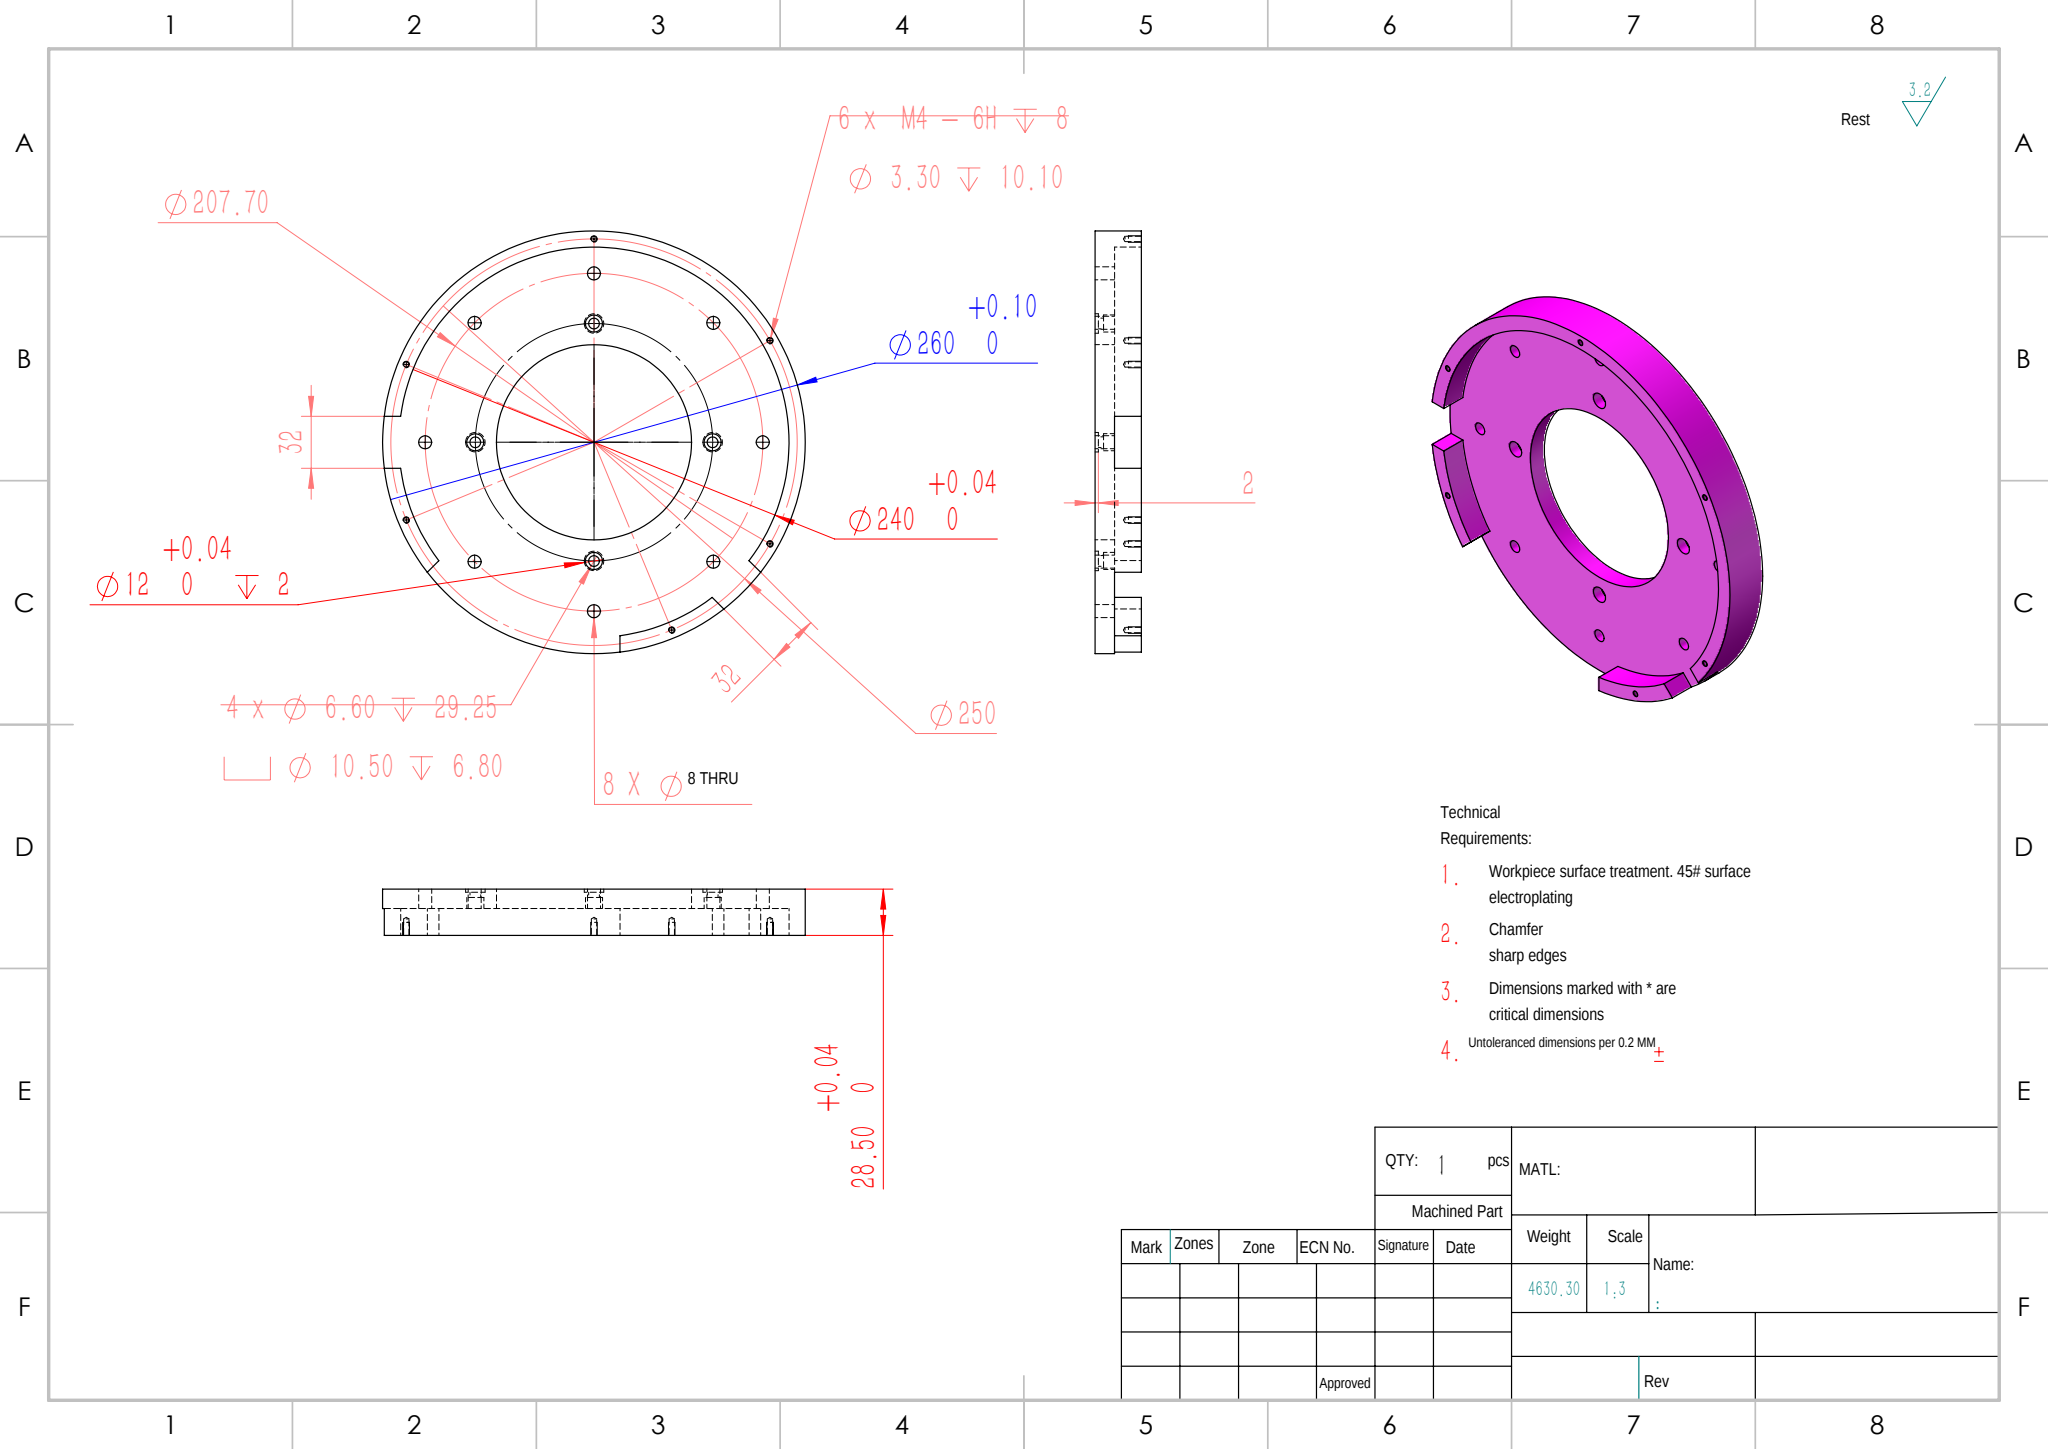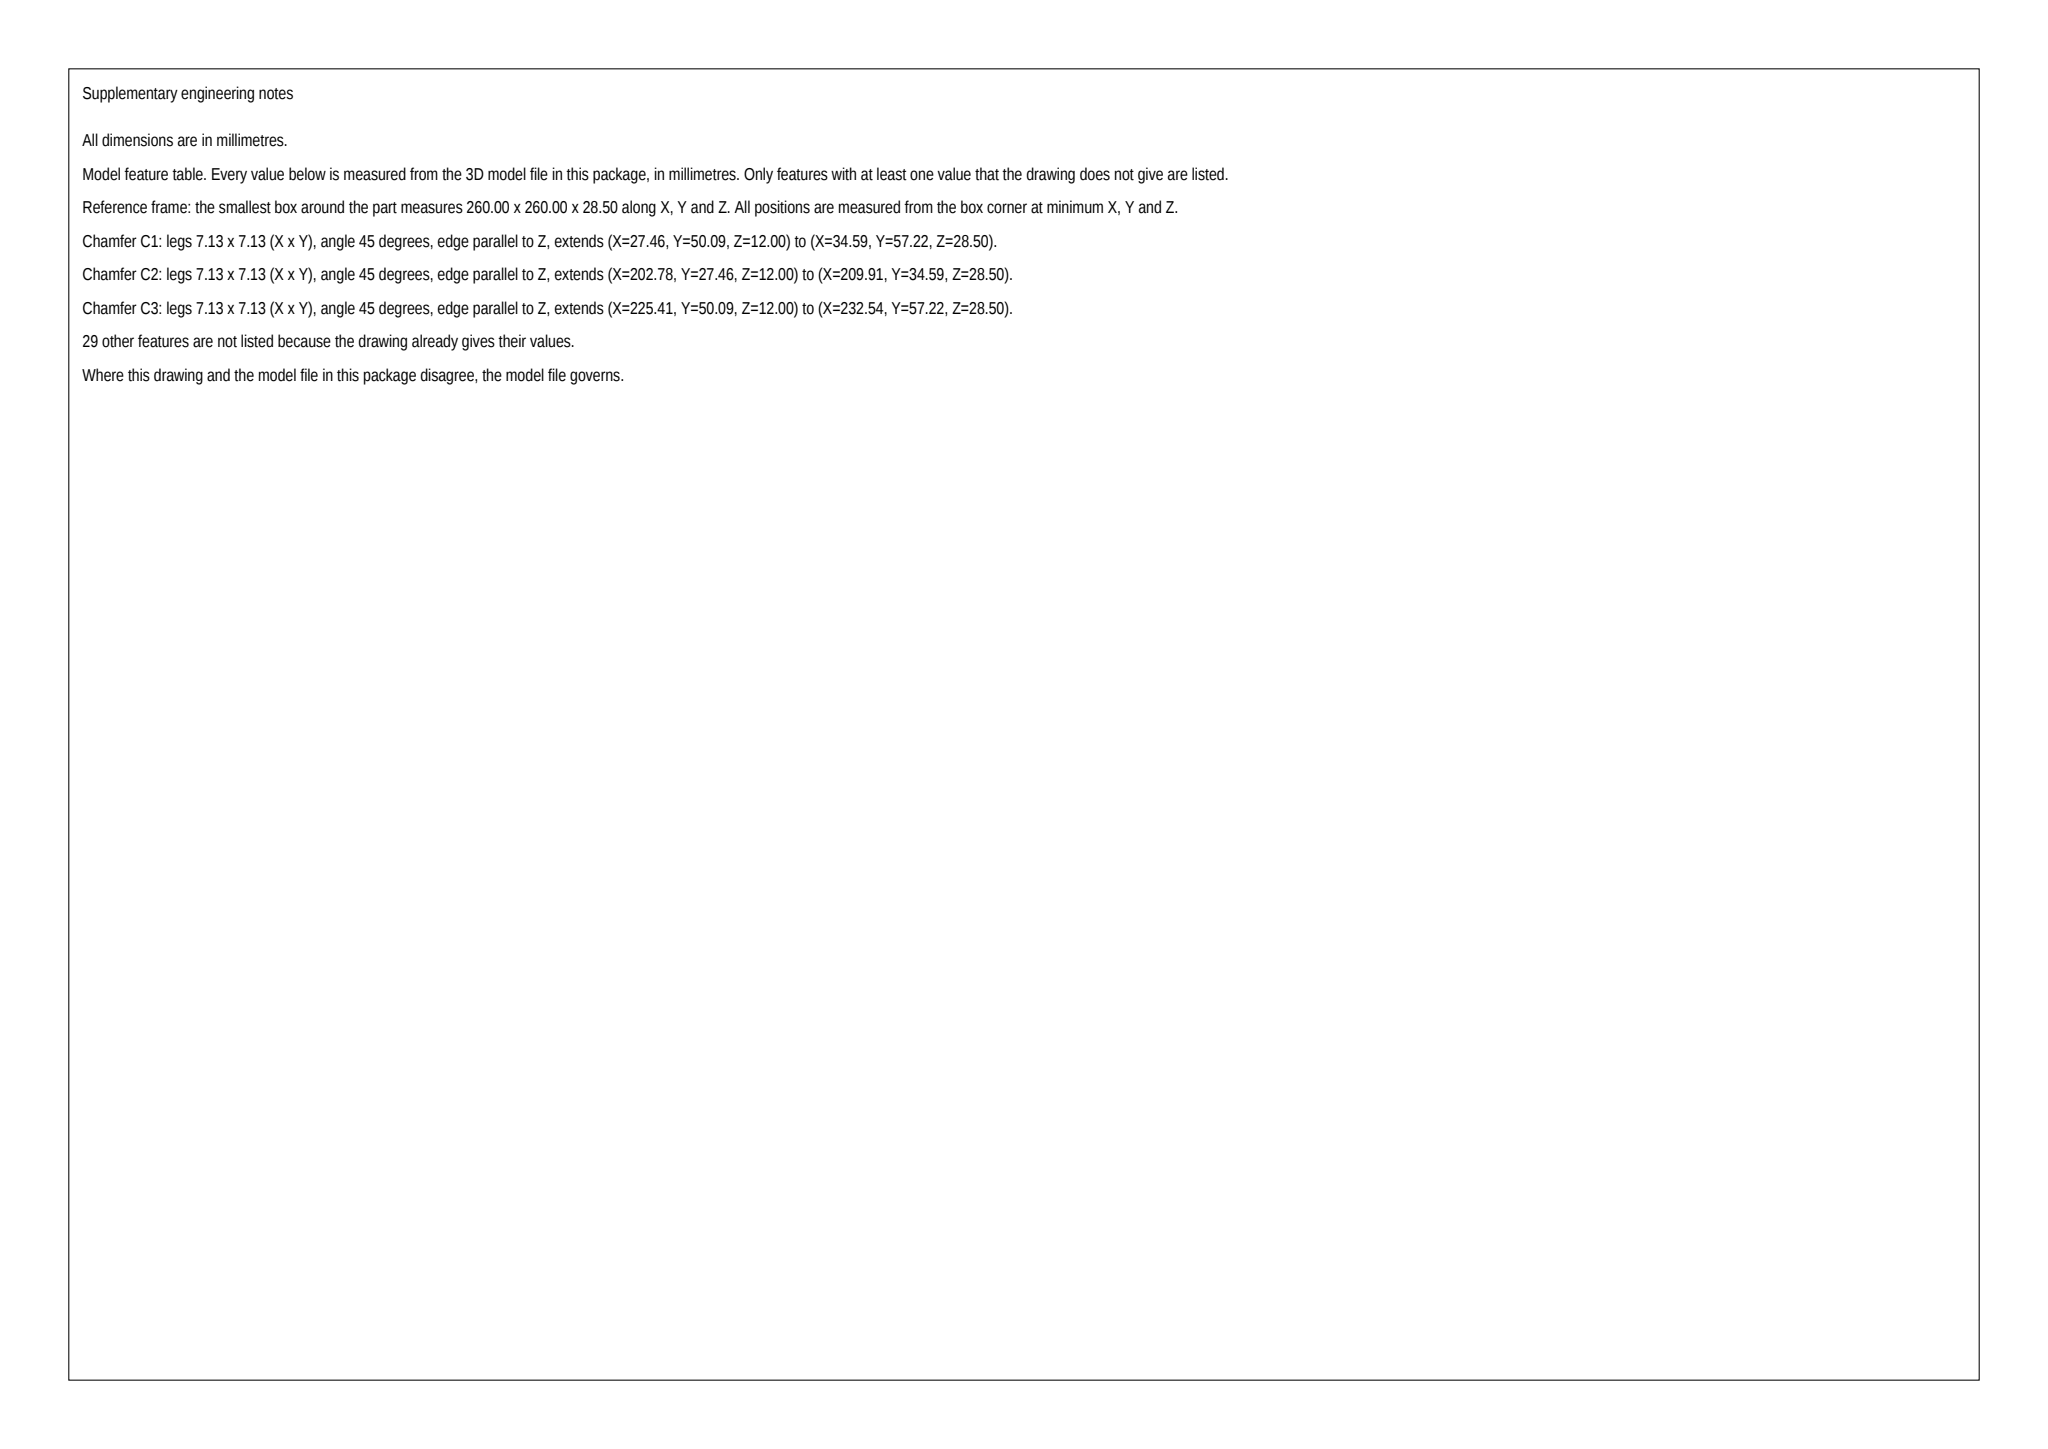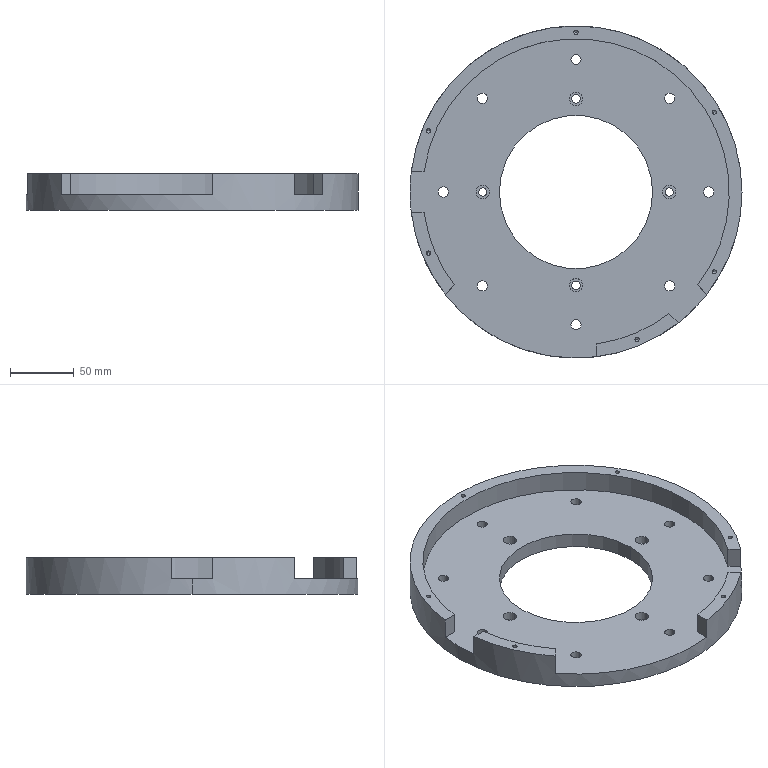Part | SolidWorks | mm | 1 solid | 90 faces | box 260 x 260 x 28.5 mm | volume 589848 mm3 | cylinder 59 | plane 19 | cone 12 | commonest cylinder face diameters 8 x16 3.3 x12 12 x8 10.5 x8 6.6 x8 240 x3 120 x2 260 x2
build123d program:
from build123d import *

# Parameters (mm, degrees)
SKETCH1_R                                         = 130
SKETCH1_R_2                                       = 60
BOSS_EXTRUDE1_DEPTH                               = 12
SKETCH2_R                                         = 130
SKETCH2_R_2                                       = 120
BOSS_EXTRUDE2_DEPTH                               = 16.5
HOLE_SIZE_ACCORDING_TO_HEXAGON_SOCKET_D           = 6.6
HOLE_SIZE_ACCORDING_TO_HEXAGON_SOCKET_DEPTH       = 29.25
HOLE_SIZE_ACCORDING_TO_HEXAGON_SOCKET_CBORE_D     = 10.5
HOLE_SIZE_ACCORDING_TO_HEXAGON_SOCKET_CBORE_DEPTH = 6.8
HOLE_SIZE_ACCORDING_TO_HEXAGON_SOCKET_TIP         = 1.983
SKETCH5_R                                         = 6
CUT_EXTRUDE1_DEPTH                                = 2
SKETCH6_R                                         = 4
CUT_EXTRUDE2_DEPTH                                = 13
CUT_EXTRUDE3_DEPTH                                = 16.5
SKETCH8_W                                         = 75
SKETCH8_H                                         = 75
CUT_EXTRUDE4_DEPTH                                = 16.5
M4_TAPPED_HOLE1_D                                 = 3.3
M4_TAPPED_HOLE1_DEPTH                             = 10.1
M4_TAPPED_HOLE1_TIP                               = 0.9914


with BuildPart() as part:
    # Sketch1 → Boss-Extrude1 (new body)
    with BuildSketch(Plane.XY):
        Circle(SKETCH1_R)
        Circle(SKETCH1_R_2, mode=Mode.SUBTRACT)
    extrude(amount=BOSS_EXTRUDE1_DEPTH)

    # Sketch2 → Boss-Extrude2 (add)
    with BuildSketch(Plane.XY.offset(12)):
        Circle(SKETCH2_R)
        Circle(SKETCH2_R_2, mode=Mode.SUBTRACT)
    extrude(amount=BOSS_EXTRUDE2_DEPTH)

    # Hole Size _ according to_ Hexagon Socket
    with Locations(Plane.XY.offset(12)):
        with Locations((0, 73), (73, 0), (0, -73), (-73, 0), (0, 0)):
            CounterBoreHole(HOLE_SIZE_ACCORDING_TO_HEXAGON_SOCKET_D / 2, HOLE_SIZE_ACCORDING_TO_HEXAGON_SOCKET_CBORE_D / 2, HOLE_SIZE_ACCORDING_TO_HEXAGON_SOCKET_CBORE_DEPTH, depth=HOLE_SIZE_ACCORDING_TO_HEXAGON_SOCKET_DEPTH)
            with Locations((0, 0, -(HOLE_SIZE_ACCORDING_TO_HEXAGON_SOCKET_DEPTH + HOLE_SIZE_ACCORDING_TO_HEXAGON_SOCKET_TIP / 2))):  # 118° drill point
                Cone(0, HOLE_SIZE_ACCORDING_TO_HEXAGON_SOCKET_D / 2, HOLE_SIZE_ACCORDING_TO_HEXAGON_SOCKET_TIP, mode=Mode.SUBTRACT)

    # Sketch5 → Cut-Extrude1 (cut)
    with BuildSketch(Plane(origin=(0, 0, 0), x_dir=(-1, 0, 0), z_dir=(0, 0, -1))):
        with Locations((-73, 0)):
            Circle(SKETCH5_R)
        with Locations((0, -73)):
            Circle(SKETCH5_R)
        with Locations((73, 0)):
            Circle(SKETCH5_R)
        with Locations((0, 73)):
            Circle(SKETCH5_R)
    extrude(amount=-CUT_EXTRUDE1_DEPTH, mode=Mode.SUBTRACT)

    # Sketch6 → Cut-Extrude2 (cut)
    with BuildSketch(Plane.XY.offset(12)):
        with Locations((0, -103.85)):
            Circle(SKETCH6_R)
        with Locations((-73.433, -73.433)):
            Circle(SKETCH6_R)
        with Locations((-103.85, 0)):
            Circle(SKETCH6_R)
        with Locations((-73.433, 73.433)):
            Circle(SKETCH6_R)
        with Locations((0, 103.85)):
            Circle(SKETCH6_R)
        with Locations((73.433, 73.433)):
            Circle(SKETCH6_R)
        with Locations((103.85, 0)):
            Circle(SKETCH6_R)
        with Locations((73.433, -73.433)):
            Circle(SKETCH6_R)
    extrude(amount=-CUT_EXTRUDE2_DEPTH, mode=Mode.SUBTRACT)

    # Sketch7 → Cut-Extrude3 (cut)
    with BuildSketch(Plane.XY.offset(28.5)):
        with BuildLine():
            Line((-130, 16), (-115, 16))
            ThreePointArc((-115, 16), (-99, 0), (-115, -16))
            Line((-115, -16), (-130, -16))
            ThreePointArc((-130, -16), (-146, 0), (-130, 16))
        make_face()
        with BuildLine():
            Line((80.61, -103.238), (70.004, -92.631))
            ThreePointArc((70.004, -92.631), (70.004, -70.004), (92.631, -70.004))
            Line((92.631, -70.004), (103.238, -80.61))
            ThreePointArc((103.238, -80.61), (103.238, -103.238), (80.61, -103.238))
        make_face()
        with BuildLine():
            Line((-16, -130), (-16, -115))
            ThreePointArc((-16, -115), (0, -99), (16, -115))
            Line((16, -115), (16, -130))
            ThreePointArc((16, -130), (0, -146), (-16, -130))
        make_face()
        with BuildLine():
            Line((-103.238, -80.61), (-92.631, -70.004))
            ThreePointArc((-92.631, -70.004), (-70.004, -70.004), (-70.004, -92.631))
            Line((-70.004, -92.631), (-80.61, -103.238))
            ThreePointArc((-80.61, -103.238), (-103.238, -103.238), (-103.238, -80.61))
        make_face()
    extrude(amount=-CUT_EXTRUDE3_DEPTH, mode=Mode.SUBTRACT)

    # Sketch8 → Cut-Extrude4 (cut)
    with BuildSketch(Plane.XY.offset(28.5)):
        with Locations((-45.922, -110.866)):
            Rectangle(SKETCH8_W, SKETCH8_H)
    extrude(amount=-CUT_EXTRUDE4_DEPTH, mode=Mode.SUBTRACT)

    # M4 Tapped Hole1
    with Locations(Plane.XY.offset(28.5)):
        with Locations((-115.485, 47.835), (47.835, -115.485), (108.253, -62.5), (0, 125), (108.253, 62.5), (-115.485, -47.835)):
            Hole(M4_TAPPED_HOLE1_D / 2, depth=M4_TAPPED_HOLE1_DEPTH)
            with Locations((0, 0, -(M4_TAPPED_HOLE1_DEPTH + M4_TAPPED_HOLE1_TIP / 2))):  # 118° drill point
                Cone(0, M4_TAPPED_HOLE1_D / 2, M4_TAPPED_HOLE1_TIP, mode=Mode.SUBTRACT)


solid = part.part